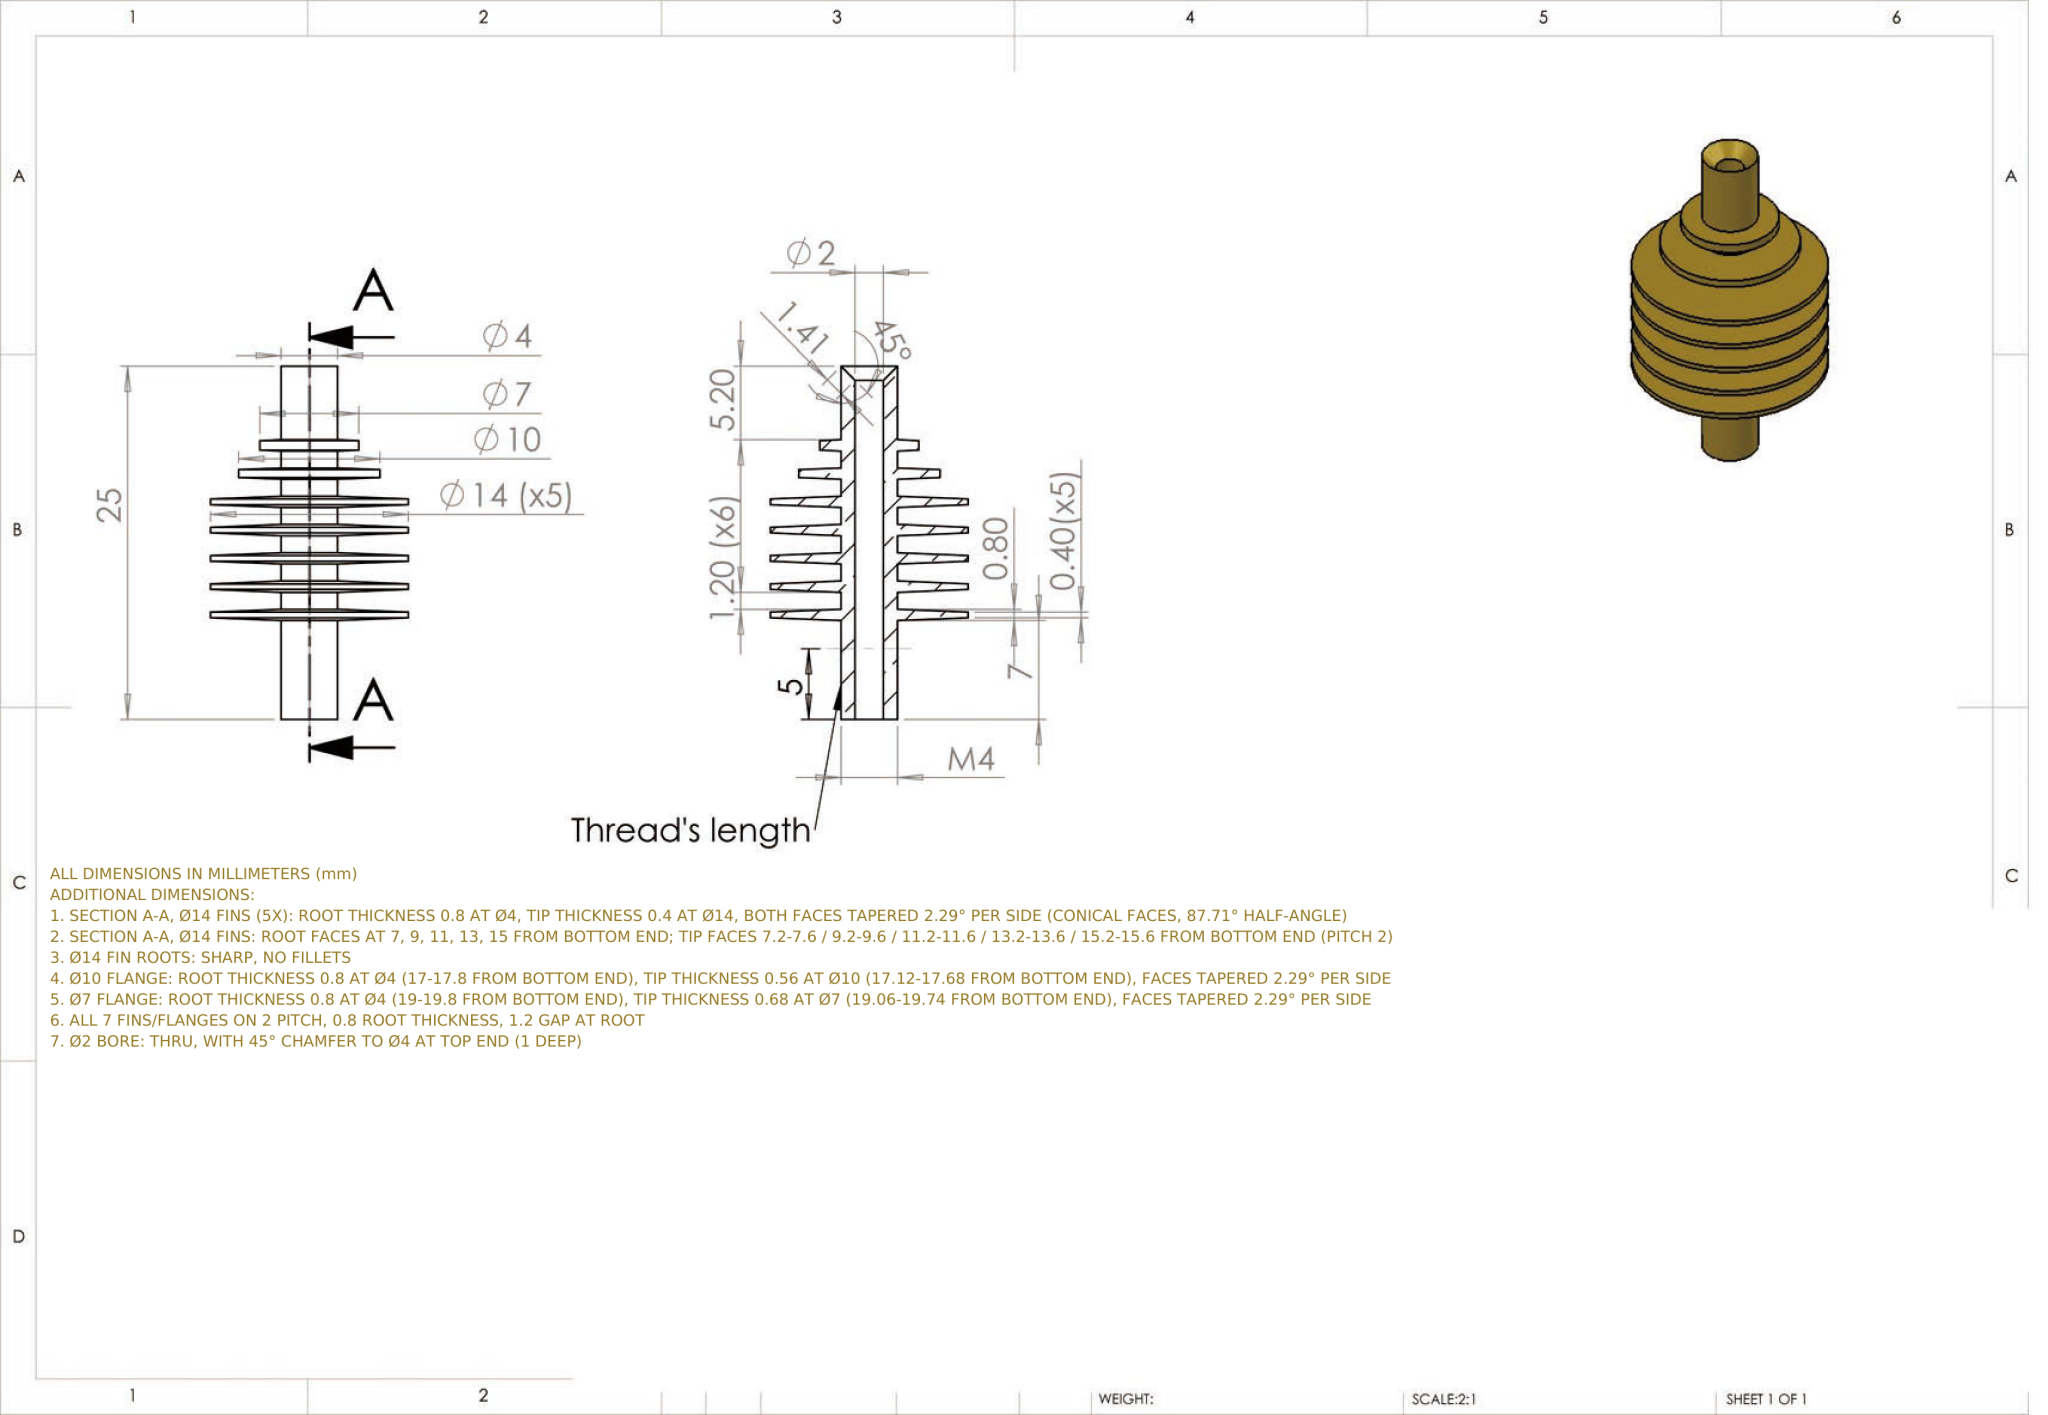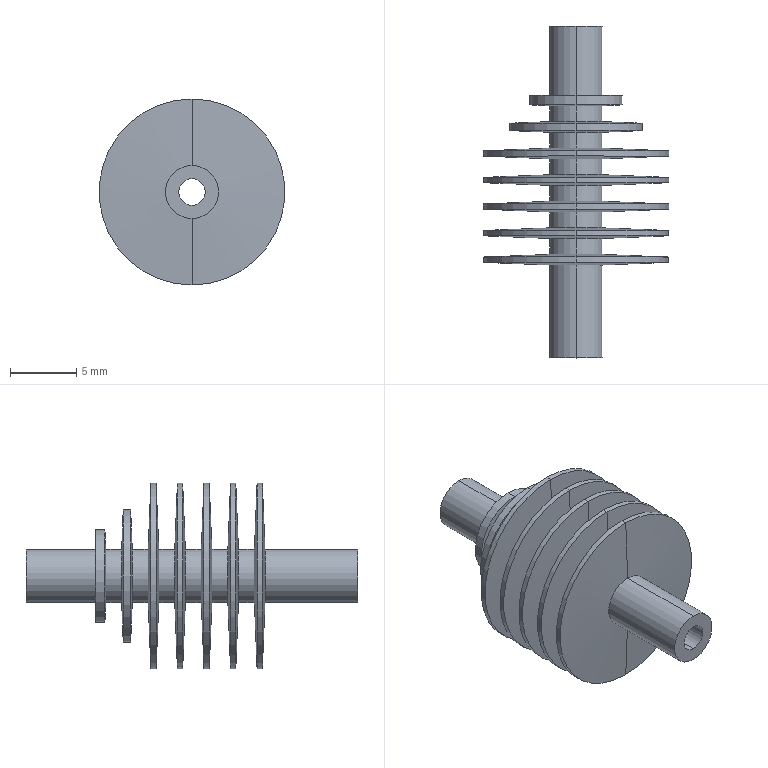Part | NX | mm | 1 solid | 63 faces | box 14 x 25 x 14 mm | volume 692 mm3 | cylinder 32 | cone 30 | plane 1 | commonest cylinder face diameters 4 x16 14 x10 7 x2 10 x2 2 x2